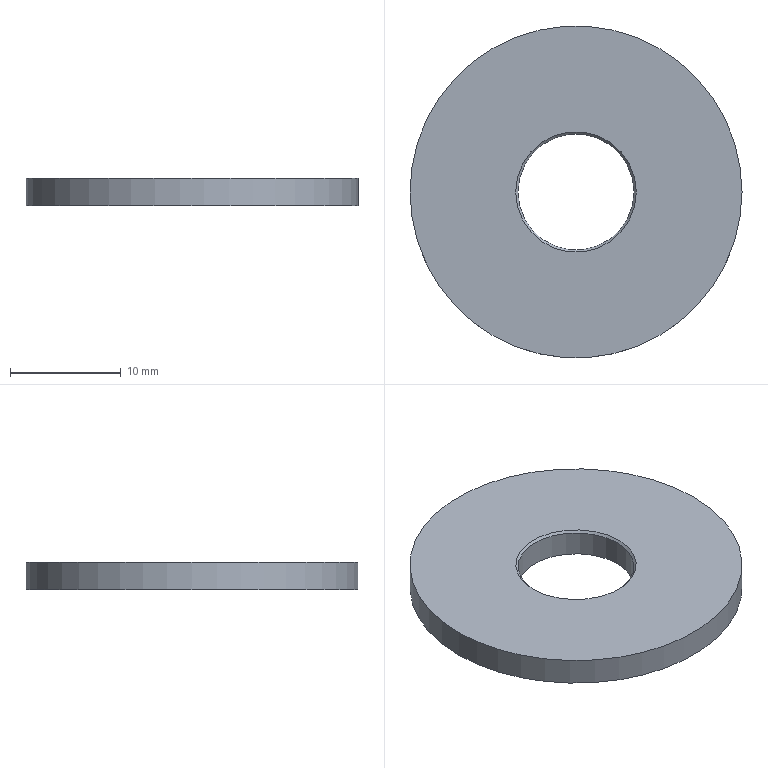Component | NX | GB-T96_1-2002_M10 | 1 solid | 5 faces | box 30 x 30 x 2.5 mm | volume 1550 mm3 | cylinder 2 | plane 2 | cone 1 | commonest cylinder face diameters 30 x1 10.5 x1
STEP:
#1=CARTESIAN_POINT('',(0.,0.,0.));
#2=DIRECTION('',(0.,0.,1.));
#3=DIRECTION('',(1.,0.,0.));
#4=AXIS2_PLACEMENT_3D('',#1,#2,#3);
#5=CARTESIAN_POINT('',(-171.087,0.,175.5));
#6=VERTEX_POINT('',#5);
#7=CARTESIAN_POINT('',(-186.087,0.,175.5));
#8=DIRECTION('',(0.,0.,1.));
#9=DIRECTION('',(1.,0.,0.));
#10=AXIS2_PLACEMENT_3D('',#7,#8,#9);
#11=CIRCLE('',#10,15.);
#12=CARTESIAN_POINT('',(-186.087,0.,175.5));
#13=DIRECTION('',(0.,0.,-1.));
#14=DIRECTION('',(-1.,0.,0.));
#15=AXIS2_PLACEMENT_3D('',#12,#13,#14);
#16=CYLINDRICAL_SURFACE('',#15,15.);
#17=CARTESIAN_POINT('',(9.425,0.));
#18=DIRECTION('',(-1.,0.));
#19=VECTOR('',#18,1.);
#20=LINE('',#17,#19);
#21=(GEOMETRIC_REPRESENTATION_CONTEXT(2)PARAMETRIC_REPRESENTATION_CONTEXT()REPRESENTATION_CONTEXT('',''));
#22=DEFINITIONAL_REPRESENTATION('',(#20),#21);
#23=PCURVE('',#16,#22);
#24=CARTESIAN_POINT('',(-186.087,0.,175.5));
#25=DIRECTION('',(0.,0.,1.));
#26=DIRECTION('',(1.,0.,0.));
#27=AXIS2_PLACEMENT_3D('',#24,#25,#26);
#28=PLANE('',#27);
#29=CARTESIAN_POINT('',(0.,0.));
#30=DIRECTION('',(1.,0.));
#31=AXIS2_PLACEMENT_2D('',#29,#30);
#32=CIRCLE('',#31,15.);
#33=(GEOMETRIC_REPRESENTATION_CONTEXT(2)PARAMETRIC_REPRESENTATION_CONTEXT()REPRESENTATION_CONTEXT('',''));
#34=DEFINITIONAL_REPRESENTATION('',(#32),#33);
#35=PCURVE('',#28,#34);
#36=SURFACE_CURVE('',#11,(#23,#35),.PCURVE_S1.);
#37=EDGE_CURVE('',#6,#6,#36,.T.);
#38=ORIENTED_EDGE('',*,*,#37,.F.);
#39=CARTESIAN_POINT('',(-171.087,0.,173.));
#40=VERTEX_POINT('',#39);
#41=CARTESIAN_POINT('',(-171.087,0.,175.5));
#42=CARTESIAN_POINT('',(-171.087,0.,173.));
#43=B_SPLINE_CURVE_WITH_KNOTS('',1,(#41,#42),.UNSPECIFIED.,.F.,.F.,(2,2),(0.,2.5),.PIECEWISE_BEZIER_KNOTS.);
#44=CARTESIAN_POINT('',(9.425,0.));
#45=DIRECTION('',(0.,1.));
#46=VECTOR('',#45,1.);
#47=LINE('',#44,#46);
#48=(GEOMETRIC_REPRESENTATION_CONTEXT(2)PARAMETRIC_REPRESENTATION_CONTEXT()REPRESENTATION_CONTEXT('',''));
#49=DEFINITIONAL_REPRESENTATION('',(#47),#48);
#50=PCURVE('',#16,#49);
#51=CARTESIAN_POINT('',(3.142,0.));
#52=DIRECTION('',(0.,1.));
#53=VECTOR('',#52,1.);
#54=LINE('',#51,#53);
#55=(GEOMETRIC_REPRESENTATION_CONTEXT(2)PARAMETRIC_REPRESENTATION_CONTEXT()REPRESENTATION_CONTEXT('',''));
#56=DEFINITIONAL_REPRESENTATION('',(#54),#55);
#57=PCURVE('',#16,#56);
#58=SEAM_CURVE('',#43,(#50,#57),.PCURVE_S1.);
#59=EDGE_CURVE('',#6,#40,#58,.T.);
#60=ORIENTED_EDGE('',*,*,#59,.T.);
#61=CARTESIAN_POINT('',(-186.087,0.,173.));
#62=DIRECTION('',(0.,0.,1.));
#63=DIRECTION('',(1.,0.,0.));
#64=AXIS2_PLACEMENT_3D('',#61,#62,#63);
#65=CIRCLE('',#64,15.);
#66=CARTESIAN_POINT('',(9.425,2.5));
#67=DIRECTION('',(-1.,0.));
#68=VECTOR('',#67,1.);
#69=LINE('',#66,#68);
#70=(GEOMETRIC_REPRESENTATION_CONTEXT(2)PARAMETRIC_REPRESENTATION_CONTEXT()REPRESENTATION_CONTEXT('',''));
#71=DEFINITIONAL_REPRESENTATION('',(#69),#70);
#72=PCURVE('',#16,#71);
#73=CARTESIAN_POINT('',(-186.087,0.,173.));
#74=DIRECTION('',(0.,0.,1.));
#75=DIRECTION('',(1.,0.,0.));
#76=AXIS2_PLACEMENT_3D('',#73,#74,#75);
#77=PLANE('',#76);
#78=CARTESIAN_POINT('',(0.,0.));
#79=DIRECTION('',(1.,0.));
#80=AXIS2_PLACEMENT_2D('',#78,#79);
#81=CIRCLE('',#80,15.);
#82=(GEOMETRIC_REPRESENTATION_CONTEXT(2)PARAMETRIC_REPRESENTATION_CONTEXT()REPRESENTATION_CONTEXT('',''));
#83=DEFINITIONAL_REPRESENTATION('',(#81),#82);
#84=PCURVE('',#77,#83);
#85=SURFACE_CURVE('',#65,(#72,#84),.PCURVE_S1.);
#86=EDGE_CURVE('',#40,#40,#85,.T.);
#87=ORIENTED_EDGE('',*,*,#86,.T.);
#88=ORIENTED_EDGE('',*,*,#59,.F.);
#89=EDGE_LOOP('',(#38,#60,#87,#88));
#90=FACE_BOUND('',#89,.T.);
#91=ADVANCED_FACE('',(#90),#16,.T.);
#92=CARTESIAN_POINT('',(-180.837,0.,175.3));
#93=VERTEX_POINT('',#92);
#94=CARTESIAN_POINT('',(-186.087,0.,175.3));
#95=DIRECTION('',(0.,0.,1.));
#96=DIRECTION('',(1.,0.,0.));
#97=AXIS2_PLACEMENT_3D('',#94,#95,#96);
#98=CIRCLE('',#97,5.25);
#99=CARTESIAN_POINT('',(-186.087,0.,175.5));
#100=DIRECTION('',(0.,0.,-1.));
#101=DIRECTION('',(-1.,0.,0.));
#102=AXIS2_PLACEMENT_3D('',#99,#100,#101);
#103=CYLINDRICAL_SURFACE('',#102,5.25);
#104=CARTESIAN_POINT('',(9.425,0.2));
#105=DIRECTION('',(-1.,0.));
#106=VECTOR('',#105,1.);
#107=LINE('',#104,#106);
#108=(GEOMETRIC_REPRESENTATION_CONTEXT(2)PARAMETRIC_REPRESENTATION_CONTEXT()REPRESENTATION_CONTEXT('',''));
#109=DEFINITIONAL_REPRESENTATION('',(#107),#108);
#110=PCURVE('',#103,#109);
#111=CARTESIAN_POINT('',(-186.087,0.,175.3));
#112=DIRECTION('',(0.,0.,1.));
#113=DIRECTION('',(1.,0.,0.));
#114=AXIS2_PLACEMENT_3D('',#111,#112,#113);
#115=CONICAL_SURFACE('',#114,5.25,0.7854);
#116=CARTESIAN_POINT('',(0.,0.));
#117=DIRECTION('',(1.,0.));
#118=VECTOR('',#117,1.);
#119=LINE('',#116,#118);
#120=(GEOMETRIC_REPRESENTATION_CONTEXT(2)PARAMETRIC_REPRESENTATION_CONTEXT()REPRESENTATION_CONTEXT('',''));
#121=DEFINITIONAL_REPRESENTATION('',(#119),#120);
#122=PCURVE('',#115,#121);
#123=SURFACE_CURVE('',#98,(#110,#122),.PCURVE_S1.);
#124=EDGE_CURVE('',#93,#93,#123,.T.);
#125=ORIENTED_EDGE('',*,*,#124,.F.);
#126=CARTESIAN_POINT('',(-180.837,0.,173.));
#127=VERTEX_POINT('',#126);
#128=CARTESIAN_POINT('',(-180.837,0.,175.3));
#129=CARTESIAN_POINT('',(-180.837,0.,173.));
#130=B_SPLINE_CURVE_WITH_KNOTS('',1,(#128,#129),.UNSPECIFIED.,.F.,.F.,(2,2),(0.2,2.5),.PIECEWISE_BEZIER_KNOTS.);
#131=CARTESIAN_POINT('',(9.425,0.));
#132=DIRECTION('',(0.,1.));
#133=VECTOR('',#132,1.);
#134=LINE('',#131,#133);
#135=(GEOMETRIC_REPRESENTATION_CONTEXT(2)PARAMETRIC_REPRESENTATION_CONTEXT()REPRESENTATION_CONTEXT('',''));
#136=DEFINITIONAL_REPRESENTATION('',(#134),#135);
#137=PCURVE('',#103,#136);
#138=CARTESIAN_POINT('',(3.142,0.));
#139=DIRECTION('',(0.,1.));
#140=VECTOR('',#139,1.);
#141=LINE('',#138,#140);
#142=(GEOMETRIC_REPRESENTATION_CONTEXT(2)PARAMETRIC_REPRESENTATION_CONTEXT()REPRESENTATION_CONTEXT('',''));
#143=DEFINITIONAL_REPRESENTATION('',(#141),#142);
#144=PCURVE('',#103,#143);
#145=SEAM_CURVE('',#130,(#137,#144),.PCURVE_S1.);
#146=EDGE_CURVE('',#93,#127,#145,.T.);
#147=ORIENTED_EDGE('',*,*,#146,.T.);
#148=CARTESIAN_POINT('',(-186.087,0.,173.));
#149=DIRECTION('',(0.,0.,1.));
#150=DIRECTION('',(1.,0.,0.));
#151=AXIS2_PLACEMENT_3D('',#148,#149,#150);
#152=CIRCLE('',#151,5.25);
#153=CARTESIAN_POINT('',(9.425,2.5));
#154=DIRECTION('',(-1.,0.));
#155=VECTOR('',#154,1.);
#156=LINE('',#153,#155);
#157=(GEOMETRIC_REPRESENTATION_CONTEXT(2)PARAMETRIC_REPRESENTATION_CONTEXT()REPRESENTATION_CONTEXT('',''));
#158=DEFINITIONAL_REPRESENTATION('',(#156),#157);
#159=PCURVE('',#103,#158);
#160=CARTESIAN_POINT('',(0.,0.));
#161=DIRECTION('',(1.,0.));
#162=AXIS2_PLACEMENT_2D('',#160,#161);
#163=CIRCLE('',#162,5.25);
#164=(GEOMETRIC_REPRESENTATION_CONTEXT(2)PARAMETRIC_REPRESENTATION_CONTEXT()REPRESENTATION_CONTEXT('',''));
#165=DEFINITIONAL_REPRESENTATION('',(#163),#164);
#166=PCURVE('',#77,#165);
#167=SURFACE_CURVE('',#152,(#159,#166),.PCURVE_S1.);
#168=EDGE_CURVE('',#127,#127,#167,.T.);
#169=ORIENTED_EDGE('',*,*,#168,.T.);
#170=ORIENTED_EDGE('',*,*,#146,.F.);
#171=EDGE_LOOP('',(#125,#147,#169,#170));
#172=FACE_BOUND('',#171,.F.);
#173=ADVANCED_FACE('',(#172),#103,.F.);
#174=CARTESIAN_POINT('',(-180.637,0.,175.5));
#175=VERTEX_POINT('',#174);
#176=CARTESIAN_POINT('',(-186.087,0.,175.5));
#177=DIRECTION('',(0.,0.,-1.));
#178=DIRECTION('',(1.,0.,0.));
#179=AXIS2_PLACEMENT_3D('',#176,#177,#178);
#180=CIRCLE('',#179,5.45);
#181=CARTESIAN_POINT('',(5.45,0.));
#182=CARTESIAN_POINT('',(5.45,-9.44));
#183=CARTESIAN_POINT('',(-2.725,-4.72));
#184=CARTESIAN_POINT('',(-10.9,-0.));
#185=CARTESIAN_POINT('',(-2.725,4.72));
#186=CARTESIAN_POINT('',(5.45,9.44));
#187=CARTESIAN_POINT('',(5.45,0.));
#188=(BOUNDED_CURVE()B_SPLINE_CURVE(2,(#181,#182,#183,#184,#185,#186,#187),.UNSPECIFIED.,.T.,.F.)B_SPLINE_CURVE_WITH_KNOTS((1,2,2,2,2,1),(-2.094,0.,2.094,4.189,6.283,8.378),.UNSPECIFIED.)CURVE()GEOMETRIC_REPRESENTATION_ITEM()RATIONAL_B_SPLINE_CURVE((1.,0.5,1.,0.5,1.,0.5,1.))REPRESENTATION_ITEM(''));
#189=(GEOMETRIC_REPRESENTATION_CONTEXT(2)PARAMETRIC_REPRESENTATION_CONTEXT()REPRESENTATION_CONTEXT('',''));
#190=DEFINITIONAL_REPRESENTATION('',(#188),#189);
#191=PCURVE('',#28,#190);
#192=CARTESIAN_POINT('',(6.283,0.2));
#193=DIRECTION('',(-1.,0.));
#194=VECTOR('',#193,1.);
#195=LINE('',#192,#194);
#196=(GEOMETRIC_REPRESENTATION_CONTEXT(2)PARAMETRIC_REPRESENTATION_CONTEXT()REPRESENTATION_CONTEXT('',''));
#197=DEFINITIONAL_REPRESENTATION('',(#195),#196);
#198=PCURVE('',#115,#197);
#199=SURFACE_CURVE('',#180,(#191,#198),.PCURVE_S1.);
#200=EDGE_CURVE('',#175,#175,#199,.T.);
#201=ORIENTED_EDGE('',*,*,#200,.T.);
#202=EDGE_LOOP('',(#201));
#203=FACE_BOUND('',#202,.T.);
#204=ORIENTED_EDGE('',*,*,#37,.T.);
#205=EDGE_LOOP('',(#204));
#206=FACE_BOUND('',#205,.T.);
#207=ADVANCED_FACE('',(#203,#206),#28,.T.);
#208=ORIENTED_EDGE('',*,*,#86,.F.);
#209=EDGE_LOOP('',(#208));
#210=FACE_BOUND('',#209,.T.);
#211=ORIENTED_EDGE('',*,*,#168,.T.);
#212=EDGE_LOOP('',(#211));
#213=FACE_BOUND('',#212,.T.);
#214=ADVANCED_FACE('',(#210,#213),#77,.F.);
#215=ORIENTED_EDGE('',*,*,#200,.T.);
#216=CARTESIAN_POINT('',(-180.837,-0.,175.3));
#217=CARTESIAN_POINT('',(-180.637,-0.,175.5));
#218=B_SPLINE_CURVE_WITH_KNOTS('',1,(#216,#217),.UNSPECIFIED.,.F.,.F.,(2,2),(0.,0.2828),.PIECEWISE_BEZIER_KNOTS.);
#219=CARTESIAN_POINT('',(0.,0.));
#220=DIRECTION('',(0.,1.));
#221=VECTOR('',#220,1.);
#222=LINE('',#219,#221);
#223=(GEOMETRIC_REPRESENTATION_CONTEXT(2)PARAMETRIC_REPRESENTATION_CONTEXT()REPRESENTATION_CONTEXT('',''));
#224=DEFINITIONAL_REPRESENTATION('',(#222),#223);
#225=PCURVE('',#115,#224);
#226=CARTESIAN_POINT('',(6.283,0.));
#227=DIRECTION('',(0.,1.));
#228=VECTOR('',#227,1.);
#229=LINE('',#226,#228);
#230=(GEOMETRIC_REPRESENTATION_CONTEXT(2)PARAMETRIC_REPRESENTATION_CONTEXT()REPRESENTATION_CONTEXT('',''));
#231=DEFINITIONAL_REPRESENTATION('',(#229),#230);
#232=PCURVE('',#115,#231);
#233=SEAM_CURVE('',#218,(#225,#232),.PCURVE_S1.);
#234=EDGE_CURVE('',#93,#175,#233,.T.);
#235=ORIENTED_EDGE('',*,*,#234,.F.);
#236=ORIENTED_EDGE('',*,*,#124,.T.);
#237=ORIENTED_EDGE('',*,*,#234,.T.);
#238=EDGE_LOOP('',(#215,#235,#236,#237));
#239=FACE_BOUND('',#238,.F.);
#240=ADVANCED_FACE('',(#239),#115,.F.);
#241=CLOSED_SHELL('',(#91,#173,#207,#214,#240));
#242=MANIFOLD_SOLID_BREP('',#241);
#243=(LENGTH_UNIT()NAMED_UNIT(*)SI_UNIT(.MILLI.,.METRE.));
#244=UNCERTAINTY_MEASURE_WITH_UNIT(LENGTH_MEASURE(0.00001),#243,'','');
#245=(NAMED_UNIT(*)PLANE_ANGLE_UNIT()SI_UNIT($,.RADIAN.));
#246=(NAMED_UNIT(*)SI_UNIT($,.STERADIAN.)SOLID_ANGLE_UNIT());
#247=(GEOMETRIC_REPRESENTATION_CONTEXT(3)GLOBAL_UNCERTAINTY_ASSIGNED_CONTEXT((#244))GLOBAL_UNIT_ASSIGNED_CONTEXT((#243,#245,#246))REPRESENTATION_CONTEXT('',''));
#248=ADVANCED_BREP_SHAPE_REPRESENTATION('',(#4,#242),#247);